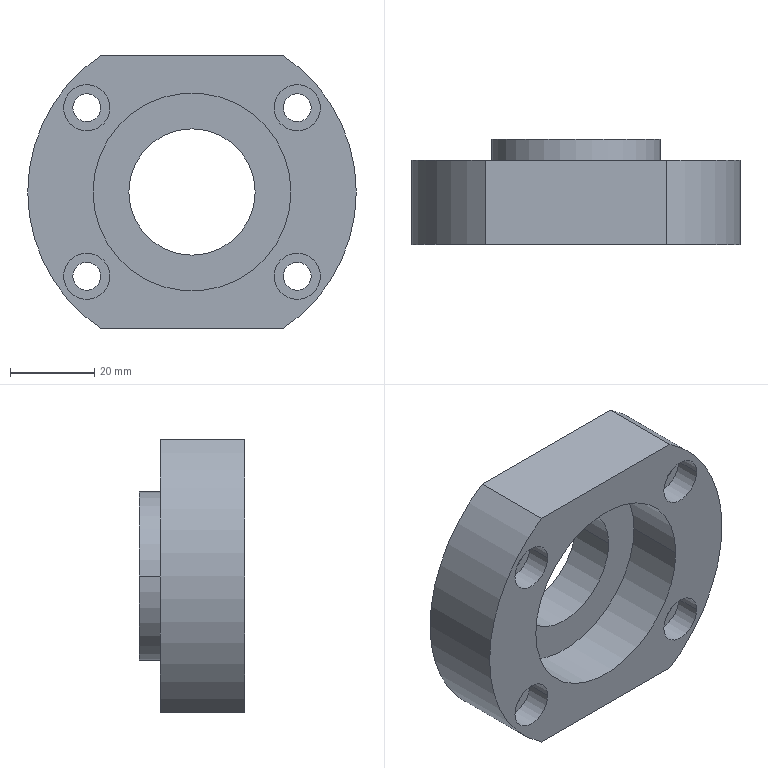Component | SolidWorks | TractionBearingHousing-3 | 1 solid | 35 faces | box 78 x 25 x 65 mm | volume 57981 mm3 | cylinder 25 | plane 10 | commonest cylinder face diameters 11 x8 6.6 x8 78 x3 47 x2 30 x2 40 x2
build123d program:
from build123d import *

# Parameters (mm, degrees)
SKETCH2_W                                       = 19.822
SKETCH2_H                                       = 75.013
EXTRUDE1_DEPTH                                  = 61.556
M6_HEX_SOCKET_HEAD_CAP_SCREW_CBORE1_D           = 6.6
M6_HEX_SOCKET_HEAD_CAP_SCREW_CBORE1_CBORE_D     = 11
M6_HEX_SOCKET_HEAD_CAP_SCREW_CBORE1_CBORE_DEPTH = 6


with BuildPart() as part:
    # Sketch1 → Revolve1 (revolve)
    with BuildSketch(Plane.XY, mode=Mode.PRIVATE) as revolve1_sk:
        Polygon((23.5, 30.807), (39, 30.807), (39, 10.807), (20, 10.807), (20, 5.807), (15, 5.807), (15, 16.807), (23.5, 16.807), align=None)
    revolve(revolve1_sk.sketch.rotate(Axis((0, -994.193, 0), (0, 1, 0)), 90), axis=Axis((0, -994.193, 0), (0, 1, 0)))

    # Sketch2 → Extrude1 (cut, through all)
    with BuildSketch(Plane(origin=(0, 30.807, 0), x_dir=(1, 0, 0), z_dir=(0, 1, 0))):
        with Locations((-42.411, -0.6478)):
            Rectangle(SKETCH2_W, SKETCH2_H)
        with Locations((42.411, -0.6478)):
            Rectangle(SKETCH2_W, SKETCH2_H)
    extrude(amount=-EXTRUDE1_DEPTH, mode=Mode.SUBTRACT)

    # M6 Hex Socket Head Cap Screw CBORE1 (through all)
    with Locations(Plane(origin=(-20, 30.807, -25), x_dir=(0, 0, 1), z_dir=(0, 1, 0))):
        with Locations((0, 0), (0, 40), (50, 40), (50, 0)):
            CounterBoreHole(M6_HEX_SOCKET_HEAD_CAP_SCREW_CBORE1_D / 2, M6_HEX_SOCKET_HEAD_CAP_SCREW_CBORE1_CBORE_D / 2, M6_HEX_SOCKET_HEAD_CAP_SCREW_CBORE1_CBORE_DEPTH)


solid = part.part

# Placed as in the assembly
solid = solid.moved(Location((385.216, 498.79, 59.606), (180, 90, 0)))
STEP:
#1=COLOUR_RGB('',0.7922,0.8196,0.9333);
#2=FILL_AREA_STYLE_COLOUR('',#1);
#3=FILL_AREA_STYLE('',(#2));
#4=SURFACE_STYLE_FILL_AREA(#3);
#5=SURFACE_SIDE_STYLE('',(#4));
#6=SURFACE_STYLE_USAGE(.BOTH.,#5);
#7=PRESENTATION_STYLE_ASSIGNMENT((#6));
#8=CARTESIAN_POINT('',(16.367,18.661,3.134));
#9=VERTEX_POINT('',#8);
#10=CARTESIAN_POINT('',(15.934,18.661,3.134));
#11=VERTEX_POINT('',#10);
#12=CARTESIAN_POINT('',(16.15,18.661,3.134));
#13=DIRECTION('',(0.,-1.,0.));
#14=DIRECTION('',(-1.,0.,0.));
#15=AXIS2_PLACEMENT_3D('',#12,#13,#14);
#16=CIRCLE('',#15,0.2165);
#17=EDGE_CURVE('',#9,#11,#16,.T.);
#18=ORIENTED_EDGE('',*,*,#17,.F.);
#19=CARTESIAN_POINT('',(16.367,18.425,3.134));
#20=VERTEX_POINT('',#19);
#21=CARTESIAN_POINT('',(16.367,18.425,3.134));
#22=DIRECTION('',(0.,-1.,0.));
#23=VECTOR('',#22,39.37);
#24=LINE('',#21,#23);
#25=EDGE_CURVE('',#9,#20,#24,.T.);
#26=ORIENTED_EDGE('',*,*,#25,.T.);
#27=CARTESIAN_POINT('',(15.934,18.425,3.134));
#28=VERTEX_POINT('',#27);
#29=CARTESIAN_POINT('',(16.15,18.425,3.134));
#30=DIRECTION('',(0.,-1.,0.));
#31=DIRECTION('',(-1.,0.,0.));
#32=AXIS2_PLACEMENT_3D('',#29,#30,#31);
#33=CIRCLE('',#32,0.2165);
#34=EDGE_CURVE('',#20,#28,#33,.T.);
#35=ORIENTED_EDGE('',*,*,#34,.T.);
#36=CARTESIAN_POINT('',(15.934,18.425,3.134));
#37=DIRECTION('',(0.,-1.,0.));
#38=VECTOR('',#37,39.37);
#39=LINE('',#36,#38);
#40=EDGE_CURVE('',#11,#28,#39,.T.);
#41=ORIENTED_EDGE('',*,*,#40,.F.);
#42=EDGE_LOOP('',(#18,#26,#35,#41));
#43=FACE_OUTER_BOUND('',#42,.T.);
#44=CARTESIAN_POINT('',(16.15,18.425,3.134));
#45=DIRECTION('',(0.,-1.,0.));
#46=DIRECTION('',(-1.,0.,0.));
#47=AXIS2_PLACEMENT_3D('',#44,#45,#46);
#48=CYLINDRICAL_SURFACE('',#47,0.2165);
#49=ADVANCED_FACE('',(#43),#48,.F.);
#50=CARTESIAN_POINT('',(16.02,19.212,3.134));
#51=VERTEX_POINT('',#50);
#52=CARTESIAN_POINT('',(16.28,19.212,3.134));
#53=VERTEX_POINT('',#52);
#54=CARTESIAN_POINT('',(16.15,19.212,3.134));
#55=DIRECTION('',(-0.,1.,-0.));
#56=DIRECTION('',(1.,0.,0.));
#57=AXIS2_PLACEMENT_3D('',#54,#55,#56);
#58=CIRCLE('',#57,0.1299);
#59=EDGE_CURVE('',#51,#53,#58,.T.);
#60=ORIENTED_EDGE('',*,*,#59,.T.);
#61=CARTESIAN_POINT('',(16.28,18.661,3.134));
#62=VERTEX_POINT('',#61);
#63=CARTESIAN_POINT('',(16.28,18.425,3.134));
#64=DIRECTION('',(0.,-1.,0.));
#65=VECTOR('',#64,39.37);
#66=LINE('',#63,#65);
#67=EDGE_CURVE('',#53,#62,#66,.T.);
#68=ORIENTED_EDGE('',*,*,#67,.T.);
#69=CARTESIAN_POINT('',(16.02,18.661,3.134));
#70=VERTEX_POINT('',#69);
#71=CARTESIAN_POINT('',(16.15,18.661,3.134));
#72=DIRECTION('',(0.,-1.,0.));
#73=DIRECTION('',(-1.,0.,0.));
#74=AXIS2_PLACEMENT_3D('',#71,#72,#73);
#75=CIRCLE('',#74,0.1299);
#76=EDGE_CURVE('',#62,#70,#75,.T.);
#77=ORIENTED_EDGE('',*,*,#76,.T.);
#78=CARTESIAN_POINT('',(16.02,18.425,3.134));
#79=DIRECTION('',(0.,-1.,0.));
#80=VECTOR('',#79,39.37);
#81=LINE('',#78,#80);
#82=EDGE_CURVE('',#51,#70,#81,.T.);
#83=ORIENTED_EDGE('',*,*,#82,.F.);
#84=EDGE_LOOP('',(#60,#68,#77,#83));
#85=FACE_OUTER_BOUND('',#84,.T.);
#86=CARTESIAN_POINT('',(16.15,18.425,3.134));
#87=DIRECTION('',(0.,-1.,0.));
#88=DIRECTION('',(-1.,0.,0.));
#89=AXIS2_PLACEMENT_3D('',#86,#87,#88);
#90=CYLINDRICAL_SURFACE('',#89,0.1299);
#91=ADVANCED_FACE('',(#85),#90,.F.);
#92=CARTESIAN_POINT('',(16.367,18.661,1.559));
#93=VERTEX_POINT('',#92);
#94=CARTESIAN_POINT('',(15.934,18.661,1.559));
#95=VERTEX_POINT('',#94);
#96=CARTESIAN_POINT('',(16.15,18.661,1.559));
#97=DIRECTION('',(0.,-1.,0.));
#98=DIRECTION('',(-1.,0.,0.));
#99=AXIS2_PLACEMENT_3D('',#96,#97,#98);
#100=CIRCLE('',#99,0.2165);
#101=EDGE_CURVE('',#93,#95,#100,.T.);
#102=ORIENTED_EDGE('',*,*,#101,.F.);
#103=CARTESIAN_POINT('',(16.367,18.425,1.559));
#104=VERTEX_POINT('',#103);
#105=CARTESIAN_POINT('',(16.367,18.425,1.559));
#106=DIRECTION('',(0.,-1.,0.));
#107=VECTOR('',#106,39.37);
#108=LINE('',#105,#107);
#109=EDGE_CURVE('',#93,#104,#108,.T.);
#110=ORIENTED_EDGE('',*,*,#109,.T.);
#111=CARTESIAN_POINT('',(15.934,18.425,1.559));
#112=VERTEX_POINT('',#111);
#113=CARTESIAN_POINT('',(16.15,18.425,1.559));
#114=DIRECTION('',(0.,-1.,0.));
#115=DIRECTION('',(-1.,0.,0.));
#116=AXIS2_PLACEMENT_3D('',#113,#114,#115);
#117=CIRCLE('',#116,0.2165);
#118=EDGE_CURVE('',#104,#112,#117,.T.);
#119=ORIENTED_EDGE('',*,*,#118,.T.);
#120=CARTESIAN_POINT('',(15.934,18.425,1.559));
#121=DIRECTION('',(0.,-1.,0.));
#122=VECTOR('',#121,39.37);
#123=LINE('',#120,#122);
#124=EDGE_CURVE('',#95,#112,#123,.T.);
#125=ORIENTED_EDGE('',*,*,#124,.F.);
#126=EDGE_LOOP('',(#102,#110,#119,#125));
#127=FACE_OUTER_BOUND('',#126,.T.);
#128=CARTESIAN_POINT('',(16.15,18.425,1.559));
#129=DIRECTION('',(0.,-1.,0.));
#130=DIRECTION('',(-1.,0.,0.));
#131=AXIS2_PLACEMENT_3D('',#128,#129,#130);
#132=CYLINDRICAL_SURFACE('',#131,0.2165);
#133=ADVANCED_FACE('',(#127),#132,.F.);
#134=CARTESIAN_POINT('',(16.02,19.212,1.559));
#135=VERTEX_POINT('',#134);
#136=CARTESIAN_POINT('',(16.28,19.212,1.559));
#137=VERTEX_POINT('',#136);
#138=CARTESIAN_POINT('',(16.15,19.212,1.559));
#139=DIRECTION('',(-0.,1.,-0.));
#140=DIRECTION('',(1.,0.,0.));
#141=AXIS2_PLACEMENT_3D('',#138,#139,#140);
#142=CIRCLE('',#141,0.1299);
#143=EDGE_CURVE('',#135,#137,#142,.T.);
#144=ORIENTED_EDGE('',*,*,#143,.T.);
#145=CARTESIAN_POINT('',(16.28,18.661,1.559));
#146=VERTEX_POINT('',#145);
#147=CARTESIAN_POINT('',(16.28,18.425,1.559));
#148=DIRECTION('',(0.,-1.,0.));
#149=VECTOR('',#148,39.37);
#150=LINE('',#147,#149);
#151=EDGE_CURVE('',#137,#146,#150,.T.);
#152=ORIENTED_EDGE('',*,*,#151,.T.);
#153=CARTESIAN_POINT('',(16.02,18.661,1.559));
#154=VERTEX_POINT('',#153);
#155=CARTESIAN_POINT('',(16.15,18.661,1.559));
#156=DIRECTION('',(0.,-1.,0.));
#157=DIRECTION('',(-1.,0.,0.));
#158=AXIS2_PLACEMENT_3D('',#155,#156,#157);
#159=CIRCLE('',#158,0.1299);
#160=EDGE_CURVE('',#146,#154,#159,.T.);
#161=ORIENTED_EDGE('',*,*,#160,.T.);
#162=CARTESIAN_POINT('',(16.02,18.425,1.559));
#163=DIRECTION('',(0.,-1.,0.));
#164=VECTOR('',#163,39.37);
#165=LINE('',#162,#164);
#166=EDGE_CURVE('',#135,#154,#165,.T.);
#167=ORIENTED_EDGE('',*,*,#166,.F.);
#168=EDGE_LOOP('',(#144,#152,#161,#167));
#169=FACE_OUTER_BOUND('',#168,.T.);
#170=CARTESIAN_POINT('',(16.15,18.425,1.559));
#171=DIRECTION('',(0.,-1.,0.));
#172=DIRECTION('',(-1.,0.,0.));
#173=AXIS2_PLACEMENT_3D('',#170,#171,#172);
#174=CYLINDRICAL_SURFACE('',#173,0.1299);
#175=ADVANCED_FACE('',(#169),#174,.F.);
#176=CARTESIAN_POINT('',(14.398,18.661,1.559));
#177=VERTEX_POINT('',#176);
#178=CARTESIAN_POINT('',(13.965,18.661,1.559));
#179=VERTEX_POINT('',#178);
#180=CARTESIAN_POINT('',(14.182,18.661,1.559));
#181=DIRECTION('',(0.,-1.,0.));
#182=DIRECTION('',(-1.,0.,0.));
#183=AXIS2_PLACEMENT_3D('',#180,#181,#182);
#184=CIRCLE('',#183,0.2165);
#185=EDGE_CURVE('',#177,#179,#184,.T.);
#186=ORIENTED_EDGE('',*,*,#185,.F.);
#187=CARTESIAN_POINT('',(14.398,18.425,1.559));
#188=VERTEX_POINT('',#187);
#189=CARTESIAN_POINT('',(14.398,18.425,1.559));
#190=DIRECTION('',(0.,-1.,0.));
#191=VECTOR('',#190,39.37);
#192=LINE('',#189,#191);
#193=EDGE_CURVE('',#177,#188,#192,.T.);
#194=ORIENTED_EDGE('',*,*,#193,.T.);
#195=CARTESIAN_POINT('',(13.965,18.425,1.559));
#196=VERTEX_POINT('',#195);
#197=CARTESIAN_POINT('',(14.182,18.425,1.559));
#198=DIRECTION('',(0.,-1.,0.));
#199=DIRECTION('',(-1.,0.,0.));
#200=AXIS2_PLACEMENT_3D('',#197,#198,#199);
#201=CIRCLE('',#200,0.2165);
#202=EDGE_CURVE('',#188,#196,#201,.T.);
#203=ORIENTED_EDGE('',*,*,#202,.T.);
#204=CARTESIAN_POINT('',(13.965,18.425,1.559));
#205=DIRECTION('',(0.,-1.,0.));
#206=VECTOR('',#205,39.37);
#207=LINE('',#204,#206);
#208=EDGE_CURVE('',#179,#196,#207,.T.);
#209=ORIENTED_EDGE('',*,*,#208,.F.);
#210=EDGE_LOOP('',(#186,#194,#203,#209));
#211=FACE_OUTER_BOUND('',#210,.T.);
#212=CARTESIAN_POINT('',(14.182,18.425,1.559));
#213=DIRECTION('',(0.,-1.,0.));
#214=DIRECTION('',(-1.,0.,0.));
#215=AXIS2_PLACEMENT_3D('',#212,#213,#214);
#216=CYLINDRICAL_SURFACE('',#215,0.2165);
#217=ADVANCED_FACE('',(#211),#216,.F.);
#218=CARTESIAN_POINT('',(14.052,19.212,1.559));
#219=VERTEX_POINT('',#218);
#220=CARTESIAN_POINT('',(14.312,19.212,1.559));
#221=VERTEX_POINT('',#220);
#222=CARTESIAN_POINT('',(14.182,19.212,1.559));
#223=DIRECTION('',(-0.,1.,-0.));
#224=DIRECTION('',(1.,0.,0.));
#225=AXIS2_PLACEMENT_3D('',#222,#223,#224);
#226=CIRCLE('',#225,0.1299);
#227=EDGE_CURVE('',#219,#221,#226,.T.);
#228=ORIENTED_EDGE('',*,*,#227,.T.);
#229=CARTESIAN_POINT('',(14.312,18.661,1.559));
#230=VERTEX_POINT('',#229);
#231=CARTESIAN_POINT('',(14.312,18.425,1.559));
#232=DIRECTION('',(0.,-1.,0.));
#233=VECTOR('',#232,39.37);
#234=LINE('',#231,#233);
#235=EDGE_CURVE('',#221,#230,#234,.T.);
#236=ORIENTED_EDGE('',*,*,#235,.T.);
#237=CARTESIAN_POINT('',(14.052,18.661,1.559));
#238=VERTEX_POINT('',#237);
#239=CARTESIAN_POINT('',(14.182,18.661,1.559));
#240=DIRECTION('',(0.,-1.,0.));
#241=DIRECTION('',(-1.,0.,0.));
#242=AXIS2_PLACEMENT_3D('',#239,#240,#241);
#243=CIRCLE('',#242,0.1299);
#244=EDGE_CURVE('',#230,#238,#243,.T.);
#245=ORIENTED_EDGE('',*,*,#244,.T.);
#246=CARTESIAN_POINT('',(14.052,18.425,1.559));
#247=DIRECTION('',(0.,-1.,0.));
#248=VECTOR('',#247,39.37);
#249=LINE('',#246,#248);
#250=EDGE_CURVE('',#219,#238,#249,.T.);
#251=ORIENTED_EDGE('',*,*,#250,.F.);
#252=EDGE_LOOP('',(#228,#236,#245,#251));
#253=FACE_OUTER_BOUND('',#252,.T.);
#254=CARTESIAN_POINT('',(14.182,18.425,1.559));
#255=DIRECTION('',(0.,-1.,0.));
#256=DIRECTION('',(-1.,0.,0.));
#257=AXIS2_PLACEMENT_3D('',#254,#255,#256);
#258=CYLINDRICAL_SURFACE('',#257,0.1299);
#259=ADVANCED_FACE('',(#253),#258,.F.);
#260=CARTESIAN_POINT('',(14.398,18.661,3.134));
#261=VERTEX_POINT('',#260);
#262=CARTESIAN_POINT('',(13.965,18.661,3.134));
#263=VERTEX_POINT('',#262);
#264=CARTESIAN_POINT('',(14.182,18.661,3.134));
#265=DIRECTION('',(0.,-1.,0.));
#266=DIRECTION('',(-1.,0.,0.));
#267=AXIS2_PLACEMENT_3D('',#264,#265,#266);
#268=CIRCLE('',#267,0.2165);
#269=EDGE_CURVE('',#261,#263,#268,.T.);
#270=ORIENTED_EDGE('',*,*,#269,.F.);
#271=CARTESIAN_POINT('',(14.398,18.425,3.134));
#272=VERTEX_POINT('',#271);
#273=CARTESIAN_POINT('',(14.398,18.425,3.134));
#274=DIRECTION('',(0.,-1.,0.));
#275=VECTOR('',#274,39.37);
#276=LINE('',#273,#275);
#277=EDGE_CURVE('',#261,#272,#276,.T.);
#278=ORIENTED_EDGE('',*,*,#277,.T.);
#279=CARTESIAN_POINT('',(13.965,18.425,3.134));
#280=VERTEX_POINT('',#279);
#281=CARTESIAN_POINT('',(14.182,18.425,3.134));
#282=DIRECTION('',(0.,-1.,0.));
#283=DIRECTION('',(-1.,0.,0.));
#284=AXIS2_PLACEMENT_3D('',#281,#282,#283);
#285=CIRCLE('',#284,0.2165);
#286=EDGE_CURVE('',#272,#280,#285,.T.);
#287=ORIENTED_EDGE('',*,*,#286,.T.);
#288=CARTESIAN_POINT('',(13.965,18.425,3.134));
#289=DIRECTION('',(0.,-1.,0.));
#290=VECTOR('',#289,39.37);
#291=LINE('',#288,#290);
#292=EDGE_CURVE('',#263,#280,#291,.T.);
#293=ORIENTED_EDGE('',*,*,#292,.F.);
#294=EDGE_LOOP('',(#270,#278,#287,#293));
#295=FACE_OUTER_BOUND('',#294,.T.);
#296=CARTESIAN_POINT('',(14.182,18.425,3.134));
#297=DIRECTION('',(0.,-1.,0.));
#298=DIRECTION('',(-1.,0.,0.));
#299=AXIS2_PLACEMENT_3D('',#296,#297,#298);
#300=CYLINDRICAL_SURFACE('',#299,0.2165);
#301=ADVANCED_FACE('',(#295),#300,.F.);
#302=CARTESIAN_POINT('',(14.052,19.212,3.134));
#303=VERTEX_POINT('',#302);
#304=CARTESIAN_POINT('',(14.312,19.212,3.134));
#305=VERTEX_POINT('',#304);
#306=CARTESIAN_POINT('',(14.182,19.212,3.134));
#307=DIRECTION('',(-0.,1.,-0.));
#308=DIRECTION('',(1.,0.,0.));
#309=AXIS2_PLACEMENT_3D('',#306,#307,#308);
#310=CIRCLE('',#309,0.1299);
#311=EDGE_CURVE('',#303,#305,#310,.T.);
#312=ORIENTED_EDGE('',*,*,#311,.T.);
#313=CARTESIAN_POINT('',(14.312,18.661,3.134));
#314=VERTEX_POINT('',#313);
#315=CARTESIAN_POINT('',(14.312,18.425,3.134));
#316=DIRECTION('',(0.,-1.,0.));
#317=VECTOR('',#316,39.37);
#318=LINE('',#315,#317);
#319=EDGE_CURVE('',#305,#314,#318,.T.);
#320=ORIENTED_EDGE('',*,*,#319,.T.);
#321=CARTESIAN_POINT('',(14.052,18.661,3.134));
#322=VERTEX_POINT('',#321);
#323=CARTESIAN_POINT('',(14.182,18.661,3.134));
#324=DIRECTION('',(0.,-1.,0.));
#325=DIRECTION('',(-1.,0.,0.));
#326=AXIS2_PLACEMENT_3D('',#323,#324,#325);
#327=CIRCLE('',#326,0.1299);
#328=EDGE_CURVE('',#314,#322,#327,.T.);
#329=ORIENTED_EDGE('',*,*,#328,.T.);
#330=CARTESIAN_POINT('',(14.052,18.425,3.134));
#331=DIRECTION('',(0.,-1.,0.));
#332=VECTOR('',#331,39.37);
#333=LINE('',#330,#332);
#334=EDGE_CURVE('',#303,#322,#333,.T.);
#335=ORIENTED_EDGE('',*,*,#334,.F.);
#336=EDGE_LOOP('',(#312,#320,#329,#335));
#337=FACE_OUTER_BOUND('',#336,.T.);
#338=CARTESIAN_POINT('',(14.182,18.425,3.134));
#339=DIRECTION('',(0.,-1.,0.));
#340=DIRECTION('',(-1.,0.,0.));
#341=AXIS2_PLACEMENT_3D('',#338,#339,#340);
#342=CYLINDRICAL_SURFACE('',#341,0.1299);
#343=ADVANCED_FACE('',(#337),#342,.F.);
#344=CARTESIAN_POINT('',(14.241,18.425,2.347));
#345=VERTEX_POINT('',#344);
#346=CARTESIAN_POINT('',(16.091,18.425,2.347));
#347=VERTEX_POINT('',#346);
#348=CARTESIAN_POINT('',(15.166,18.425,2.347));
#349=DIRECTION('',(-0.,1.,-0.));
#350=DIRECTION('',(1.,0.,0.));
#351=AXIS2_PLACEMENT_3D('',#348,#349,#350);
#352=CIRCLE('',#351,0.9252);
#353=EDGE_CURVE('',#345,#347,#352,.T.);
#354=ORIENTED_EDGE('',*,*,#353,.F.);
#355=CARTESIAN_POINT('',(14.241,18.976,2.347));
#356=VERTEX_POINT('',#355);
#357=CARTESIAN_POINT('',(14.241,58.779,2.347));
#358=DIRECTION('',(-0.,1.,-0.));
#359=VECTOR('',#358,39.37);
#360=LINE('',#357,#359);
#361=EDGE_CURVE('',#345,#356,#360,.T.);
#362=ORIENTED_EDGE('',*,*,#361,.T.);
#363=CARTESIAN_POINT('',(16.091,18.976,2.347));
#364=VERTEX_POINT('',#363);
#365=CARTESIAN_POINT('',(15.166,18.976,2.347));
#366=DIRECTION('',(-0.,1.,-0.));
#367=DIRECTION('',(1.,0.,0.));
#368=AXIS2_PLACEMENT_3D('',#365,#366,#367);
#369=CIRCLE('',#368,0.9252);
#370=EDGE_CURVE('',#356,#364,#369,.T.);
#371=ORIENTED_EDGE('',*,*,#370,.T.);
#372=CARTESIAN_POINT('',(16.091,58.779,2.347));
#373=DIRECTION('',(-0.,1.,-0.));
#374=VECTOR('',#373,39.37);
#375=LINE('',#372,#374);
#376=EDGE_CURVE('',#347,#364,#375,.T.);
#377=ORIENTED_EDGE('',*,*,#376,.F.);
#378=EDGE_LOOP('',(#354,#362,#371,#377));
#379=FACE_OUTER_BOUND('',#378,.T.);
#380=CARTESIAN_POINT('',(15.166,58.779,2.347));
#381=DIRECTION('',(-0.,1.,-0.));
#382=DIRECTION('',(1.,0.,0.));
#383=AXIS2_PLACEMENT_3D('',#380,#381,#382);
#384=CYLINDRICAL_SURFACE('',#383,0.9252);
#385=ADVANCED_FACE('',(#379),#384,.F.);
#386=CARTESIAN_POINT('',(14.575,18.976,2.347));
#387=VERTEX_POINT('',#386);
#388=CARTESIAN_POINT('',(15.757,18.976,2.347));
#389=VERTEX_POINT('',#388);
#390=CARTESIAN_POINT('',(15.166,18.976,2.347));
#391=DIRECTION('',(-0.,1.,-0.));
#392=DIRECTION('',(1.,0.,0.));
#393=AXIS2_PLACEMENT_3D('',#390,#391,#392);
#394=CIRCLE('',#393,0.5906);
#395=EDGE_CURVE('',#387,#389,#394,.T.);
#396=ORIENTED_EDGE('',*,*,#395,.F.);
#397=CARTESIAN_POINT('',(14.575,19.409,2.347));
#398=VERTEX_POINT('',#397);
#399=CARTESIAN_POINT('',(14.575,58.779,2.347));
#400=DIRECTION('',(-0.,1.,-0.));
#401=VECTOR('',#400,39.37);
#402=LINE('',#399,#401);
#403=EDGE_CURVE('',#387,#398,#402,.T.);
#404=ORIENTED_EDGE('',*,*,#403,.T.);
#405=CARTESIAN_POINT('',(15.757,19.409,2.347));
#406=VERTEX_POINT('',#405);
#407=CARTESIAN_POINT('',(15.166,19.409,2.347));
#408=DIRECTION('',(-0.,1.,-0.));
#409=DIRECTION('',(1.,0.,0.));
#410=AXIS2_PLACEMENT_3D('',#407,#408,#409);
#411=CIRCLE('',#410,0.5906);
#412=EDGE_CURVE('',#398,#406,#411,.T.);
#413=ORIENTED_EDGE('',*,*,#412,.T.);
#414=CARTESIAN_POINT('',(15.757,58.779,2.347));
#415=DIRECTION('',(-0.,1.,-0.));
#416=VECTOR('',#415,39.37);
#417=LINE('',#414,#416);
#418=EDGE_CURVE('',#389,#406,#417,.T.);
#419=ORIENTED_EDGE('',*,*,#418,.F.);
#420=EDGE_LOOP('',(#396,#404,#413,#419));
#421=FACE_OUTER_BOUND('',#420,.T.);
#422=CARTESIAN_POINT('',(15.166,58.779,2.347));
#423=DIRECTION('',(-0.,1.,-0.));
#424=DIRECTION('',(1.,0.,0.));
#425=AXIS2_PLACEMENT_3D('',#422,#423,#424);
#426=CYLINDRICAL_SURFACE('',#425,0.5906);
#427=ADVANCED_FACE('',(#421),#426,.F.);
#428=CARTESIAN_POINT('',(15.953,19.212,2.347));
#429=VERTEX_POINT('',#428);
#430=CARTESIAN_POINT('',(14.379,19.212,2.347));
#431=VERTEX_POINT('',#430);
#432=CARTESIAN_POINT('',(15.166,19.212,2.347));
#433=DIRECTION('',(-0.,1.,-0.));
#434=DIRECTION('',(1.,0.,0.));
#435=AXIS2_PLACEMENT_3D('',#432,#433,#434);
#436=CIRCLE('',#435,0.7874);
#437=EDGE_CURVE('',#429,#431,#436,.T.);
#438=ORIENTED_EDGE('',*,*,#437,.T.);
#439=CARTESIAN_POINT('',(14.379,19.409,2.347));
#440=VERTEX_POINT('',#439);
#441=CARTESIAN_POINT('',(14.379,58.779,2.347));
#442=DIRECTION('',(-0.,1.,-0.));
#443=VECTOR('',#442,39.37);
#444=LINE('',#441,#443);
#445=EDGE_CURVE('',#431,#440,#444,.T.);
#446=ORIENTED_EDGE('',*,*,#445,.T.);
#447=CARTESIAN_POINT('',(15.953,19.409,2.347));
#448=VERTEX_POINT('',#447);
#449=CARTESIAN_POINT('',(15.166,19.409,2.347));
#450=DIRECTION('',(-0.,1.,-0.));
#451=DIRECTION('',(1.,0.,0.));
#452=AXIS2_PLACEMENT_3D('',#449,#450,#451);
#453=CIRCLE('',#452,0.7874);
#454=EDGE_CURVE('',#448,#440,#453,.T.);
#455=ORIENTED_EDGE('',*,*,#454,.F.);
#456=CARTESIAN_POINT('',(15.953,58.779,2.347));
#457=DIRECTION('',(-0.,1.,-0.));
#458=VECTOR('',#457,39.37);
#459=LINE('',#456,#458);
#460=EDGE_CURVE('',#429,#448,#459,.T.);
#461=ORIENTED_EDGE('',*,*,#460,.F.);
#462=EDGE_LOOP('',(#438,#446,#455,#461));
#463=FACE_OUTER_BOUND('',#462,.T.);
#464=CARTESIAN_POINT('',(15.166,58.779,2.347));
#465=DIRECTION('',(-0.,1.,-0.));
#466=DIRECTION('',(1.,0.,0.));
#467=AXIS2_PLACEMENT_3D('',#464,#465,#466);
#468=CYLINDRICAL_SURFACE('',#467,0.7874);
#469=ADVANCED_FACE('',(#463),#468,.T.);
#470=CARTESIAN_POINT('',(16.015,18.425,3.626));
#471=VERTEX_POINT('',#470);
#472=CARTESIAN_POINT('',(16.701,18.425,2.347));
#473=VERTEX_POINT('',#472);
#474=CARTESIAN_POINT('',(15.166,18.425,2.347));
#475=DIRECTION('',(-0.,1.,-0.));
#476=DIRECTION('',(1.,0.,0.));
#477=AXIS2_PLACEMENT_3D('',#474,#475,#476);
#478=CIRCLE('',#477,1.535);
#479=EDGE_CURVE('',#471,#473,#478,.T.);
#480=ORIENTED_EDGE('',*,*,#479,.T.);
#481=CARTESIAN_POINT('',(16.701,19.212,2.347));
#482=VERTEX_POINT('',#481);
#483=CARTESIAN_POINT('',(16.701,58.779,2.347));
#484=DIRECTION('',(-0.,1.,-0.));
#485=VECTOR('',#484,39.37);
#486=LINE('',#483,#485);
#487=EDGE_CURVE('',#473,#482,#486,.T.);
#488=ORIENTED_EDGE('',*,*,#487,.T.);
#489=CARTESIAN_POINT('',(16.015,19.212,3.626));
#490=VERTEX_POINT('',#489);
#491=CARTESIAN_POINT('',(15.166,19.212,2.347));
#492=DIRECTION('',(-0.,1.,-0.));
#493=DIRECTION('',(1.,0.,0.));
#494=AXIS2_PLACEMENT_3D('',#491,#492,#493);
#495=CIRCLE('',#494,1.535);
#496=EDGE_CURVE('',#490,#482,#495,.T.);
#497=ORIENTED_EDGE('',*,*,#496,.F.);
#498=CARTESIAN_POINT('',(16.015,58.779,3.626));
#499=DIRECTION('',(-0.,1.,-0.));
#500=VECTOR('',#499,39.37);
#501=LINE('',#498,#500);
#502=EDGE_CURVE('',#471,#490,#501,.T.);
#503=ORIENTED_EDGE('',*,*,#502,.F.);
#504=EDGE_LOOP('',(#480,#488,#497,#503));
#505=FACE_OUTER_BOUND('',#504,.T.);
#506=CARTESIAN_POINT('',(15.166,58.779,2.347));
#507=DIRECTION('',(-0.,1.,-0.));
#508=DIRECTION('',(1.,0.,0.));
#509=AXIS2_PLACEMENT_3D('',#506,#507,#508);
#510=CYLINDRICAL_SURFACE('',#509,1.535);
#511=ADVANCED_FACE('',(#505),#510,.T.);
#512=ORIENTED_EDGE('',*,*,#487,.F.);
#513=CARTESIAN_POINT('',(16.015,18.425,1.067));
#514=VERTEX_POINT('',#513);
#515=CARTESIAN_POINT('',(15.166,18.425,2.347));
#516=DIRECTION('',(-0.,1.,-0.));
#517=DIRECTION('',(1.,0.,0.));
#518=AXIS2_PLACEMENT_3D('',#515,#516,#517);
#519=CIRCLE('',#518,1.535);
#520=EDGE_CURVE('',#473,#514,#519,.T.);
#521=ORIENTED_EDGE('',*,*,#520,.T.);
#522=CARTESIAN_POINT('',(16.015,19.212,1.067));
#523=VERTEX_POINT('',#522);
#524=CARTESIAN_POINT('',(16.015,58.779,1.067));
#525=DIRECTION('',(0.,-1.,0.));
#526=VECTOR('',#525,39.37);
#527=LINE('',#524,#526);
#528=EDGE_CURVE('',#523,#514,#527,.T.);
#529=ORIENTED_EDGE('',*,*,#528,.F.);
#530=CARTESIAN_POINT('',(15.166,19.212,2.347));
#531=DIRECTION('',(-0.,1.,-0.));
#532=DIRECTION('',(1.,0.,0.));
#533=AXIS2_PLACEMENT_3D('',#530,#531,#532);
#534=CIRCLE('',#533,1.535);
#535=EDGE_CURVE('',#482,#523,#534,.T.);
#536=ORIENTED_EDGE('',*,*,#535,.F.);
#537=EDGE_LOOP('',(#512,#521,#529,#536));
#538=FACE_OUTER_BOUND('',#537,.T.);
#539=CARTESIAN_POINT('',(15.166,58.779,2.347));
#540=DIRECTION('',(-0.,1.,-0.));
#541=DIRECTION('',(1.,0.,0.));
#542=AXIS2_PLACEMENT_3D('',#539,#540,#541);
#543=CYLINDRICAL_SURFACE('',#542,1.535);
#544=ADVANCED_FACE('',(#538),#543,.T.);
#545=CARTESIAN_POINT('',(14.317,18.425,1.067));
#546=VERTEX_POINT('',#545);
#547=CARTESIAN_POINT('',(14.317,19.212,1.067));
#548=VERTEX_POINT('',#547);
#549=CARTESIAN_POINT('',(14.317,58.779,1.067));
#550=DIRECTION('',(-0.,1.,-0.));
#551=VECTOR('',#550,39.37);
#552=LINE('',#549,#551);
#553=EDGE_CURVE('',#546,#548,#552,.T.);
#554=ORIENTED_EDGE('',*,*,#553,.F.);
#555=CARTESIAN_POINT('',(14.317,18.425,3.626));
#556=VERTEX_POINT('',#555);
#557=CARTESIAN_POINT('',(15.166,18.425,2.347));
#558=DIRECTION('',(-0.,1.,-0.));
#559=DIRECTION('',(1.,0.,0.));
#560=AXIS2_PLACEMENT_3D('',#557,#558,#559);
#561=CIRCLE('',#560,1.535);
#562=EDGE_CURVE('',#546,#556,#561,.T.);
#563=ORIENTED_EDGE('',*,*,#562,.T.);
#564=CARTESIAN_POINT('',(14.317,19.212,3.626));
#565=VERTEX_POINT('',#564);
#566=CARTESIAN_POINT('',(14.317,58.779,3.626));
#567=DIRECTION('',(0.,-1.,0.));
#568=VECTOR('',#567,39.37);
#569=LINE('',#566,#568);
#570=EDGE_CURVE('',#565,#556,#569,.T.);
#571=ORIENTED_EDGE('',*,*,#570,.F.);
#572=CARTESIAN_POINT('',(15.166,19.212,2.347));
#573=DIRECTION('',(-0.,1.,-0.));
#574=DIRECTION('',(1.,0.,0.));
#575=AXIS2_PLACEMENT_3D('',#572,#573,#574);
#576=CIRCLE('',#575,1.535);
#577=EDGE_CURVE('',#548,#565,#576,.T.);
#578=ORIENTED_EDGE('',*,*,#577,.F.);
#579=EDGE_LOOP('',(#554,#563,#571,#578));
#580=FACE_OUTER_BOUND('',#579,.T.);
#581=CARTESIAN_POINT('',(15.166,58.779,2.347));
#582=DIRECTION('',(-0.,1.,-0.));
#583=DIRECTION('',(1.,0.,0.));
#584=AXIS2_PLACEMENT_3D('',#581,#582,#583);
#585=CYLINDRICAL_SURFACE('',#584,1.535);
#586=ADVANCED_FACE('',(#580),#585,.T.);
#587=ORIENTED_EDGE('',*,*,#59,.F.);
#588=CARTESIAN_POINT('',(16.15,19.212,3.134));
#589=DIRECTION('',(-0.,1.,-0.));
#590=DIRECTION('',(1.,0.,0.));
#591=AXIS2_PLACEMENT_3D('',#588,#589,#590);
#592=CIRCLE('',#591,0.1299);
#593=EDGE_CURVE('',#53,#51,#592,.T.);
#594=ORIENTED_EDGE('',*,*,#593,.F.);
#595=EDGE_LOOP('',(#587,#594));
#596=FACE_BOUND('',#595,.T.);
#597=ORIENTED_EDGE('',*,*,#143,.F.);
#598=CARTESIAN_POINT('',(16.15,19.212,1.559));
#599=DIRECTION('',(-0.,1.,-0.));
#600=DIRECTION('',(1.,0.,0.));
#601=AXIS2_PLACEMENT_3D('',#598,#599,#600);
#602=CIRCLE('',#601,0.1299);
#603=EDGE_CURVE('',#137,#135,#602,.T.);
#604=ORIENTED_EDGE('',*,*,#603,.F.);
#605=EDGE_LOOP('',(#597,#604));
#606=FACE_BOUND('',#605,.T.);
#607=ORIENTED_EDGE('',*,*,#227,.F.);
#608=CARTESIAN_POINT('',(14.182,19.212,1.559));
#609=DIRECTION('',(-0.,1.,-0.));
#610=DIRECTION('',(1.,0.,0.));
#611=AXIS2_PLACEMENT_3D('',#608,#609,#610);
#612=CIRCLE('',#611,0.1299);
#613=EDGE_CURVE('',#221,#219,#612,.T.);
#614=ORIENTED_EDGE('',*,*,#613,.F.);
#615=EDGE_LOOP('',(#607,#614));
#616=FACE_BOUND('',#615,.T.);
#617=ORIENTED_EDGE('',*,*,#311,.F.);
#618=CARTESIAN_POINT('',(14.182,19.212,3.134));
#619=DIRECTION('',(-0.,1.,-0.));
#620=DIRECTION('',(1.,0.,0.));
#621=AXIS2_PLACEMENT_3D('',#618,#619,#620);
#622=CIRCLE('',#621,0.1299);
#623=EDGE_CURVE('',#305,#303,#622,.T.);
#624=ORIENTED_EDGE('',*,*,#623,.F.);
#625=EDGE_LOOP('',(#617,#624));
#626=FACE_BOUND('',#625,.T.);
#627=CARTESIAN_POINT('',(15.166,19.212,1.067));
#628=DIRECTION('',(1.,0.,-0.));
#629=VECTOR('',#628,39.37);
#630=LINE('',#627,#629);
#631=EDGE_CURVE('',#548,#523,#630,.T.);
#632=ORIENTED_EDGE('',*,*,#631,.F.);
#633=ORIENTED_EDGE('',*,*,#577,.T.);
#634=CARTESIAN_POINT('',(15.166,19.212,3.626));
#635=DIRECTION('',(-1.,-0.,-0.));
#636=VECTOR('',#635,39.37);
#637=LINE('',#634,#636);
#638=EDGE_CURVE('',#490,#565,#637,.T.);
#639=ORIENTED_EDGE('',*,*,#638,.F.);
#640=ORIENTED_EDGE('',*,*,#496,.T.);
#641=ORIENTED_EDGE('',*,*,#535,.T.);
#642=EDGE_LOOP('',(#632,#633,#639,#640,#641));
#643=FACE_OUTER_BOUND('',#642,.T.);
#644=ORIENTED_EDGE('',*,*,#437,.F.);
#645=CARTESIAN_POINT('',(15.166,19.212,2.347));
#646=DIRECTION('',(-0.,1.,-0.));
#647=DIRECTION('',(1.,0.,0.));
#648=AXIS2_PLACEMENT_3D('',#645,#646,#647);
#649=CIRCLE('',#648,0.7874);
#650=EDGE_CURVE('',#431,#429,#649,.T.);
#651=ORIENTED_EDGE('',*,*,#650,.F.);
#652=EDGE_LOOP('',(#644,#651));
#653=FACE_BOUND('',#652,.T.);
#654=CARTESIAN_POINT('',(15.166,19.212,0.8113));
#655=DIRECTION('',(-0.,1.,-0.));
#656=DIRECTION('',(1.,0.,-0.));
#657=AXIS2_PLACEMENT_3D('',#654,#655,#656);
#658=PLANE('',#657);
#659=ADVANCED_FACE('',(#596,#606,#616,#626,#643,#653),#658,.T.);
#660=ORIENTED_EDGE('',*,*,#445,.F.);
#661=ORIENTED_EDGE('',*,*,#650,.T.);
#662=ORIENTED_EDGE('',*,*,#460,.T.);
#663=CARTESIAN_POINT('',(15.166,19.409,2.347));
#664=DIRECTION('',(-0.,1.,-0.));
#665=DIRECTION('',(1.,0.,0.));
#666=AXIS2_PLACEMENT_3D('',#663,#664,#665);
#667=CIRCLE('',#666,0.7874);
#668=EDGE_CURVE('',#440,#448,#667,.T.);
#669=ORIENTED_EDGE('',*,*,#668,.F.);
#670=EDGE_LOOP('',(#660,#661,#662,#669));
#671=FACE_OUTER_BOUND('',#670,.T.);
#672=CARTESIAN_POINT('',(15.166,58.779,2.347));
#673=DIRECTION('',(-0.,1.,-0.));
#674=DIRECTION('',(1.,0.,0.));
#675=AXIS2_PLACEMENT_3D('',#672,#673,#674);
#676=CYLINDRICAL_SURFACE('',#675,0.7874);
#677=ADVANCED_FACE('',(#671),#676,.T.);
#678=ORIENTED_EDGE('',*,*,#454,.T.);
#679=ORIENTED_EDGE('',*,*,#668,.T.);
#680=EDGE_LOOP('',(#678,#679));
#681=FACE_OUTER_BOUND('',#680,.T.);
#682=CARTESIAN_POINT('',(15.166,19.409,2.347));
#683=DIRECTION('',(-0.,1.,-0.));
#684=DIRECTION('',(1.,0.,0.));
#685=AXIS2_PLACEMENT_3D('',#682,#683,#684);
#686=CIRCLE('',#685,0.5906);
#687=EDGE_CURVE('',#406,#398,#686,.T.);
#688=ORIENTED_EDGE('',*,*,#687,.F.);
#689=ORIENTED_EDGE('',*,*,#412,.F.);
#690=EDGE_LOOP('',(#688,#689));
#691=FACE_BOUND('',#690,.T.);
#692=CARTESIAN_POINT('',(15.166,19.409,1.559));
#693=DIRECTION('',(-0.,1.,-0.));
#694=DIRECTION('',(1.,0.,-0.));
#695=AXIS2_PLACEMENT_3D('',#692,#693,#694);
#696=PLANE('',#695);
#697=ADVANCED_FACE('',(#681,#691),#696,.T.);
#698=ORIENTED_EDGE('',*,*,#403,.F.);
#699=CARTESIAN_POINT('',(15.166,18.976,2.347));
#700=DIRECTION('',(-0.,1.,-0.));
#701=DIRECTION('',(1.,0.,0.));
#702=AXIS2_PLACEMENT_3D('',#699,#700,#701);
#703=CIRCLE('',#702,0.5906);
#704=EDGE_CURVE('',#389,#387,#703,.T.);
#705=ORIENTED_EDGE('',*,*,#704,.F.);
#706=ORIENTED_EDGE('',*,*,#418,.T.);
#707=ORIENTED_EDGE('',*,*,#687,.T.);
#708=EDGE_LOOP('',(#698,#705,#706,#707));
#709=FACE_OUTER_BOUND('',#708,.T.);
#710=CARTESIAN_POINT('',(15.166,58.779,2.347));
#711=DIRECTION('',(-0.,1.,-0.));
#712=DIRECTION('',(1.,0.,0.));
#713=AXIS2_PLACEMENT_3D('',#710,#711,#712);
#714=CYLINDRICAL_SURFACE('',#713,0.5906);
#715=ADVANCED_FACE('',(#709),#714,.F.);
#716=ORIENTED_EDGE('',*,*,#704,.T.);
#717=ORIENTED_EDGE('',*,*,#395,.T.);
#718=EDGE_LOOP('',(#716,#717));
#719=FACE_BOUND('',#718,.T.);
#720=CARTESIAN_POINT('',(15.166,18.976,2.347));
#721=DIRECTION('',(-0.,1.,-0.));
#722=DIRECTION('',(1.,0.,0.));
#723=AXIS2_PLACEMENT_3D('',#720,#721,#722);
#724=CIRCLE('',#723,0.9252);
#725=EDGE_CURVE('',#364,#356,#724,.T.);
#726=ORIENTED_EDGE('',*,*,#725,.F.);
#727=ORIENTED_EDGE('',*,*,#370,.F.);
#728=EDGE_LOOP('',(#726,#727));
#729=FACE_OUTER_BOUND('',#728,.T.);
#730=CARTESIAN_POINT('',(15.166,18.976,1.421));
#731=DIRECTION('',(0.,-1.,0.));
#732=DIRECTION('',(-1.,-0.,0.));
#733=AXIS2_PLACEMENT_3D('',#730,#731,#732);
#734=PLANE('',#733);
#735=ADVANCED_FACE('',(#719,#729),#734,.T.);
#736=ORIENTED_EDGE('',*,*,#361,.F.);
#737=CARTESIAN_POINT('',(15.166,18.425,2.347));
#738=DIRECTION('',(-0.,1.,-0.));
#739=DIRECTION('',(1.,0.,0.));
#740=AXIS2_PLACEMENT_3D('',#737,#738,#739);
#741=CIRCLE('',#740,0.9252);
#742=EDGE_CURVE('',#347,#345,#741,.T.);
#743=ORIENTED_EDGE('',*,*,#742,.F.);
#744=ORIENTED_EDGE('',*,*,#376,.T.);
#745=ORIENTED_EDGE('',*,*,#725,.T.);
#746=EDGE_LOOP('',(#736,#743,#744,#745));
#747=FACE_OUTER_BOUND('',#746,.T.);
#748=CARTESIAN_POINT('',(15.166,58.779,2.347));
#749=DIRECTION('',(-0.,1.,-0.));
#750=DIRECTION('',(1.,0.,0.));
#751=AXIS2_PLACEMENT_3D('',#748,#749,#750);
#752=CYLINDRICAL_SURFACE('',#751,0.9252);
#753=ADVANCED_FACE('',(#747),#752,.F.);
#754=CARTESIAN_POINT('',(16.15,18.425,3.134));
#755=DIRECTION('',(0.,-1.,0.));
#756=DIRECTION('',(-1.,0.,0.));
#757=AXIS2_PLACEMENT_3D('',#754,#755,#756);
#758=CIRCLE('',#757,0.2165);
#759=EDGE_CURVE('',#28,#20,#758,.T.);
#760=ORIENTED_EDGE('',*,*,#759,.F.);
#761=ORIENTED_EDGE('',*,*,#34,.F.);
#762=EDGE_LOOP('',(#760,#761));
#763=FACE_BOUND('',#762,.T.);
#764=CARTESIAN_POINT('',(16.15,18.425,1.559));
#765=DIRECTION('',(0.,-1.,0.));
#766=DIRECTION('',(-1.,0.,0.));
#767=AXIS2_PLACEMENT_3D('',#764,#765,#766);
#768=CIRCLE('',#767,0.2165);
#769=EDGE_CURVE('',#112,#104,#768,.T.);
#770=ORIENTED_EDGE('',*,*,#769,.F.);
#771=ORIENTED_EDGE('',*,*,#118,.F.);
#772=EDGE_LOOP('',(#770,#771));
#773=FACE_BOUND('',#772,.T.);
#774=CARTESIAN_POINT('',(14.182,18.425,1.559));
#775=DIRECTION('',(0.,-1.,0.));
#776=DIRECTION('',(-1.,0.,0.));
#777=AXIS2_PLACEMENT_3D('',#774,#775,#776);
#778=CIRCLE('',#777,0.2165);
#779=EDGE_CURVE('',#196,#188,#778,.T.);
#780=ORIENTED_EDGE('',*,*,#779,.F.);
#781=ORIENTED_EDGE('',*,*,#202,.F.);
#782=EDGE_LOOP('',(#780,#781));
#783=FACE_BOUND('',#782,.T.);
#784=CARTESIAN_POINT('',(14.182,18.425,3.134));
#785=DIRECTION('',(0.,-1.,0.));
#786=DIRECTION('',(-1.,0.,0.));
#787=AXIS2_PLACEMENT_3D('',#784,#785,#786);
#788=CIRCLE('',#787,0.2165);
#789=EDGE_CURVE('',#280,#272,#788,.T.);
#790=ORIENTED_EDGE('',*,*,#789,.F.);
#791=ORIENTED_EDGE('',*,*,#286,.F.);
#792=EDGE_LOOP('',(#790,#791));
#793=FACE_BOUND('',#792,.T.);
#794=CARTESIAN_POINT('',(15.166,18.425,1.067));
#795=DIRECTION('',(-1.,-0.,0.));
#796=VECTOR('',#795,39.37);
#797=LINE('',#794,#796);
#798=EDGE_CURVE('',#514,#546,#797,.T.);
#799=ORIENTED_EDGE('',*,*,#798,.F.);
#800=ORIENTED_EDGE('',*,*,#520,.F.);
#801=ORIENTED_EDGE('',*,*,#479,.F.);
#802=CARTESIAN_POINT('',(15.166,18.425,3.626));
#803=DIRECTION('',(1.,0.,0.));
#804=VECTOR('',#803,39.37);
#805=LINE('',#802,#804);
#806=EDGE_CURVE('',#556,#471,#805,.T.);
#807=ORIENTED_EDGE('',*,*,#806,.F.);
#808=ORIENTED_EDGE('',*,*,#562,.F.);
#809=EDGE_LOOP('',(#799,#800,#801,#807,#808));
#810=FACE_OUTER_BOUND('',#809,.T.);
#811=ORIENTED_EDGE('',*,*,#742,.T.);
#812=ORIENTED_EDGE('',*,*,#353,.T.);
#813=EDGE_LOOP('',(#811,#812));
#814=FACE_BOUND('',#813,.T.);
#815=CARTESIAN_POINT('',(15.166,18.425,1.421));
#816=DIRECTION('',(0.,-1.,0.));
#817=DIRECTION('',(-1.,-0.,0.));
#818=AXIS2_PLACEMENT_3D('',#815,#816,#817);
#819=PLANE('',#818);
#820=ADVANCED_FACE('',(#763,#773,#783,#793,#810,#814),#819,.T.);
#821=ORIENTED_EDGE('',*,*,#570,.T.);
#822=ORIENTED_EDGE('',*,*,#806,.T.);
#823=ORIENTED_EDGE('',*,*,#502,.T.);
#824=ORIENTED_EDGE('',*,*,#638,.T.);
#825=EDGE_LOOP('',(#821,#822,#823,#824));
#826=FACE_OUTER_BOUND('',#825,.T.);
#827=CARTESIAN_POINT('',(16.617,19.409,3.626));
#828=DIRECTION('',(0.,-0.,-1.));
#829=DIRECTION('',(1.,0.,0.));
#830=AXIS2_PLACEMENT_3D('',#827,#828,#829);
#831=PLANE('',#830);
#832=ADVANCED_FACE('',(#826),#831,.F.);
#833=ORIENTED_EDGE('',*,*,#528,.T.);
#834=ORIENTED_EDGE('',*,*,#798,.T.);
#835=ORIENTED_EDGE('',*,*,#553,.T.);
#836=ORIENTED_EDGE('',*,*,#631,.T.);
#837=EDGE_LOOP('',(#833,#834,#835,#836));
#838=FACE_OUTER_BOUND('',#837,.T.);
#839=CARTESIAN_POINT('',(16.617,19.409,1.067));
#840=DIRECTION('',(0.,0.,1.));
#841=DIRECTION('',(-1.,-0.,0.));
#842=AXIS2_PLACEMENT_3D('',#839,#840,#841);
#843=PLANE('',#842);
#844=ADVANCED_FACE('',(#838),#843,.F.);
#845=ORIENTED_EDGE('',*,*,#319,.F.);
#846=ORIENTED_EDGE('',*,*,#623,.T.);
#847=ORIENTED_EDGE('',*,*,#334,.T.);
#848=CARTESIAN_POINT('',(14.182,18.661,3.134));
#849=DIRECTION('',(0.,-1.,0.));
#850=DIRECTION('',(-1.,0.,0.));
#851=AXIS2_PLACEMENT_3D('',#848,#849,#850);
#852=CIRCLE('',#851,0.1299);
#853=EDGE_CURVE('',#322,#314,#852,.T.);
#854=ORIENTED_EDGE('',*,*,#853,.T.);
#855=EDGE_LOOP('',(#845,#846,#847,#854));
#856=FACE_OUTER_BOUND('',#855,.T.);
#857=CARTESIAN_POINT('',(14.182,18.425,3.134));
#858=DIRECTION('',(0.,-1.,0.));
#859=DIRECTION('',(-1.,0.,0.));
#860=AXIS2_PLACEMENT_3D('',#857,#858,#859);
#861=CYLINDRICAL_SURFACE('',#860,0.1299);
#862=ADVANCED_FACE('',(#856),#861,.F.);
#863=ORIENTED_EDGE('',*,*,#853,.F.);
#864=ORIENTED_EDGE('',*,*,#328,.F.);
#865=EDGE_LOOP('',(#863,#864));
#866=FACE_BOUND('',#865,.T.);
#867=CARTESIAN_POINT('',(14.182,18.661,3.134));
#868=DIRECTION('',(0.,-1.,0.));
#869=DIRECTION('',(-1.,0.,0.));
#870=AXIS2_PLACEMENT_3D('',#867,#868,#869);
#871=CIRCLE('',#870,0.2165);
#872=EDGE_CURVE('',#263,#261,#871,.T.);
#873=ORIENTED_EDGE('',*,*,#872,.T.);
#874=ORIENTED_EDGE('',*,*,#269,.T.);
#875=EDGE_LOOP('',(#873,#874));
#876=FACE_OUTER_BOUND('',#875,.T.);
#877=CARTESIAN_POINT('',(14.182,18.661,3.004));
#878=DIRECTION('',(-0.,1.,-0.));
#879=DIRECTION('',(1.,0.,-0.));
#880=AXIS2_PLACEMENT_3D('',#877,#878,#879);
#881=PLANE('',#880);
#882=ADVANCED_FACE('',(#866,#876),#881,.F.);
#883=ORIENTED_EDGE('',*,*,#277,.F.);
#884=ORIENTED_EDGE('',*,*,#872,.F.);
#885=ORIENTED_EDGE('',*,*,#292,.T.);
#886=ORIENTED_EDGE('',*,*,#789,.T.);
#887=EDGE_LOOP('',(#883,#884,#885,#886));
#888=FACE_OUTER_BOUND('',#887,.T.);
#889=CARTESIAN_POINT('',(14.182,18.425,3.134));
#890=DIRECTION('',(0.,-1.,0.));
#891=DIRECTION('',(-1.,0.,0.));
#892=AXIS2_PLACEMENT_3D('',#889,#890,#891);
#893=CYLINDRICAL_SURFACE('',#892,0.2165);
#894=ADVANCED_FACE('',(#888),#893,.F.);
#895=ORIENTED_EDGE('',*,*,#235,.F.);
#896=ORIENTED_EDGE('',*,*,#613,.T.);
#897=ORIENTED_EDGE('',*,*,#250,.T.);
#898=CARTESIAN_POINT('',(14.182,18.661,1.559));
#899=DIRECTION('',(0.,-1.,0.));
#900=DIRECTION('',(-1.,0.,0.));
#901=AXIS2_PLACEMENT_3D('',#898,#899,#900);
#902=CIRCLE('',#901,0.1299);
#903=EDGE_CURVE('',#238,#230,#902,.T.);
#904=ORIENTED_EDGE('',*,*,#903,.T.);
#905=EDGE_LOOP('',(#895,#896,#897,#904));
#906=FACE_OUTER_BOUND('',#905,.T.);
#907=CARTESIAN_POINT('',(14.182,18.425,1.559));
#908=DIRECTION('',(0.,-1.,0.));
#909=DIRECTION('',(-1.,0.,0.));
#910=AXIS2_PLACEMENT_3D('',#907,#908,#909);
#911=CYLINDRICAL_SURFACE('',#910,0.1299);
#912=ADVANCED_FACE('',(#906),#911,.F.);
#913=ORIENTED_EDGE('',*,*,#903,.F.);
#914=ORIENTED_EDGE('',*,*,#244,.F.);
#915=EDGE_LOOP('',(#913,#914));
#916=FACE_BOUND('',#915,.T.);
#917=CARTESIAN_POINT('',(14.182,18.661,1.559));
#918=DIRECTION('',(0.,-1.,0.));
#919=DIRECTION('',(-1.,0.,0.));
#920=AXIS2_PLACEMENT_3D('',#917,#918,#919);
#921=CIRCLE('',#920,0.2165);
#922=EDGE_CURVE('',#179,#177,#921,.T.);
#923=ORIENTED_EDGE('',*,*,#922,.T.);
#924=ORIENTED_EDGE('',*,*,#185,.T.);
#925=EDGE_LOOP('',(#923,#924));
#926=FACE_OUTER_BOUND('',#925,.T.);
#927=CARTESIAN_POINT('',(14.182,18.661,1.429));
#928=DIRECTION('',(-0.,1.,-0.));
#929=DIRECTION('',(1.,0.,-0.));
#930=AXIS2_PLACEMENT_3D('',#927,#928,#929);
#931=PLANE('',#930);
#932=ADVANCED_FACE('',(#916,#926),#931,.F.);
#933=ORIENTED_EDGE('',*,*,#193,.F.);
#934=ORIENTED_EDGE('',*,*,#922,.F.);
#935=ORIENTED_EDGE('',*,*,#208,.T.);
#936=ORIENTED_EDGE('',*,*,#779,.T.);
#937=EDGE_LOOP('',(#933,#934,#935,#936));
#938=FACE_OUTER_BOUND('',#937,.T.);
#939=CARTESIAN_POINT('',(14.182,18.425,1.559));
#940=DIRECTION('',(0.,-1.,0.));
#941=DIRECTION('',(-1.,0.,0.));
#942=AXIS2_PLACEMENT_3D('',#939,#940,#941);
#943=CYLINDRICAL_SURFACE('',#942,0.2165);
#944=ADVANCED_FACE('',(#938),#943,.F.);
#945=ORIENTED_EDGE('',*,*,#151,.F.);
#946=ORIENTED_EDGE('',*,*,#603,.T.);
#947=ORIENTED_EDGE('',*,*,#166,.T.);
#948=CARTESIAN_POINT('',(16.15,18.661,1.559));
#949=DIRECTION('',(0.,-1.,0.));
#950=DIRECTION('',(-1.,0.,0.));
#951=AXIS2_PLACEMENT_3D('',#948,#949,#950);
#952=CIRCLE('',#951,0.1299);
#953=EDGE_CURVE('',#154,#146,#952,.T.);
#954=ORIENTED_EDGE('',*,*,#953,.T.);
#955=EDGE_LOOP('',(#945,#946,#947,#954));
#956=FACE_OUTER_BOUND('',#955,.T.);
#957=CARTESIAN_POINT('',(16.15,18.425,1.559));
#958=DIRECTION('',(0.,-1.,0.));
#959=DIRECTION('',(-1.,0.,0.));
#960=AXIS2_PLACEMENT_3D('',#957,#958,#959);
#961=CYLINDRICAL_SURFACE('',#960,0.1299);
#962=ADVANCED_FACE('',(#956),#961,.F.);
#963=ORIENTED_EDGE('',*,*,#953,.F.);
#964=ORIENTED_EDGE('',*,*,#160,.F.);
#965=EDGE_LOOP('',(#963,#964));
#966=FACE_BOUND('',#965,.T.);
#967=CARTESIAN_POINT('',(16.15,18.661,1.559));
#968=DIRECTION('',(0.,-1.,0.));
#969=DIRECTION('',(-1.,0.,0.));
#970=AXIS2_PLACEMENT_3D('',#967,#968,#969);
#971=CIRCLE('',#970,0.2165);
#972=EDGE_CURVE('',#95,#93,#971,.T.);
#973=ORIENTED_EDGE('',*,*,#972,.T.);
#974=ORIENTED_EDGE('',*,*,#101,.T.);
#975=EDGE_LOOP('',(#973,#974));
#976=FACE_OUTER_BOUND('',#975,.T.);
#977=CARTESIAN_POINT('',(16.15,18.661,1.429));
#978=DIRECTION('',(-0.,1.,-0.));
#979=DIRECTION('',(1.,0.,-0.));
#980=AXIS2_PLACEMENT_3D('',#977,#978,#979);
#981=PLANE('',#980);
#982=ADVANCED_FACE('',(#966,#976),#981,.F.);
#983=ORIENTED_EDGE('',*,*,#109,.F.);
#984=ORIENTED_EDGE('',*,*,#972,.F.);
#985=ORIENTED_EDGE('',*,*,#124,.T.);
#986=ORIENTED_EDGE('',*,*,#769,.T.);
#987=EDGE_LOOP('',(#983,#984,#985,#986));
#988=FACE_OUTER_BOUND('',#987,.T.);
#989=CARTESIAN_POINT('',(16.15,18.425,1.559));
#990=DIRECTION('',(0.,-1.,0.));
#991=DIRECTION('',(-1.,0.,0.));
#992=AXIS2_PLACEMENT_3D('',#989,#990,#991);
#993=CYLINDRICAL_SURFACE('',#992,0.2165);
#994=ADVANCED_FACE('',(#988),#993,.F.);
#995=ORIENTED_EDGE('',*,*,#67,.F.);
#996=ORIENTED_EDGE('',*,*,#593,.T.);
#997=ORIENTED_EDGE('',*,*,#82,.T.);
#998=CARTESIAN_POINT('',(16.15,18.661,3.134));
#999=DIRECTION('',(0.,-1.,0.));
#1000=DIRECTION('',(-1.,0.,0.));
#1001=AXIS2_PLACEMENT_3D('',#998,#999,#1000);
#1002=CIRCLE('',#1001,0.1299);
#1003=EDGE_CURVE('',#70,#62,#1002,.T.);
#1004=ORIENTED_EDGE('',*,*,#1003,.T.);
#1005=EDGE_LOOP('',(#995,#996,#997,#1004));
#1006=FACE_OUTER_BOUND('',#1005,.T.);
#1007=CARTESIAN_POINT('',(16.15,18.425,3.134));
#1008=DIRECTION('',(0.,-1.,0.));
#1009=DIRECTION('',(-1.,0.,0.));
#1010=AXIS2_PLACEMENT_3D('',#1007,#1008,#1009);
#1011=CYLINDRICAL_SURFACE('',#1010,0.1299);
#1012=ADVANCED_FACE('',(#1006),#1011,.F.);
#1013=ORIENTED_EDGE('',*,*,#1003,.F.);
#1014=ORIENTED_EDGE('',*,*,#76,.F.);
#1015=EDGE_LOOP('',(#1013,#1014));
#1016=FACE_BOUND('',#1015,.T.);
#1017=CARTESIAN_POINT('',(16.15,18.661,3.134));
#1018=DIRECTION('',(0.,-1.,0.));
#1019=DIRECTION('',(-1.,0.,0.));
#1020=AXIS2_PLACEMENT_3D('',#1017,#1018,#1019);
#1021=CIRCLE('',#1020,0.2165);
#1022=EDGE_CURVE('',#11,#9,#1021,.T.);
#1023=ORIENTED_EDGE('',*,*,#1022,.T.);
#1024=ORIENTED_EDGE('',*,*,#17,.T.);
#1025=EDGE_LOOP('',(#1023,#1024));
#1026=FACE_OUTER_BOUND('',#1025,.T.);
#1027=CARTESIAN_POINT('',(16.15,18.661,3.004));
#1028=DIRECTION('',(-0.,1.,-0.));
#1029=DIRECTION('',(1.,0.,-0.));
#1030=AXIS2_PLACEMENT_3D('',#1027,#1028,#1029);
#1031=PLANE('',#1030);
#1032=ADVANCED_FACE('',(#1016,#1026),#1031,.F.);
#1033=ORIENTED_EDGE('',*,*,#25,.F.);
#1034=ORIENTED_EDGE('',*,*,#1022,.F.);
#1035=ORIENTED_EDGE('',*,*,#40,.T.);
#1036=ORIENTED_EDGE('',*,*,#759,.T.);
#1037=EDGE_LOOP('',(#1033,#1034,#1035,#1036));
#1038=FACE_OUTER_BOUND('',#1037,.T.);
#1039=CARTESIAN_POINT('',(16.15,18.425,3.134));
#1040=DIRECTION('',(0.,-1.,0.));
#1041=DIRECTION('',(-1.,0.,0.));
#1042=AXIS2_PLACEMENT_3D('',#1039,#1040,#1041);
#1043=CYLINDRICAL_SURFACE('',#1042,0.2165);
#1044=ADVANCED_FACE('',(#1038),#1043,.F.);
#1045=CLOSED_SHELL('',(#49,#91,#133,#175,#217,#259,#301,#343,#385,#427,#469,#511,#544,#586,#659,#677,#697,#715,#735,#753,#820,#832,#844,#862,#882,#894,#912,#932,#944,#962,#982,#994,#1012,#1032,#1044));
#1046=MANIFOLD_SOLID_BREP('',#1045);
#1047=STYLED_ITEM('',(#7),#1046);
#1048=(LENGTH_UNIT()NAMED_UNIT(*)SI_UNIT($,.METRE.));
#1049=LENGTH_MEASURE_WITH_UNIT(LENGTH_MEASURE(0.0254),#1048);
#1050=DIMENSIONAL_EXPONENTS(1.,0.,0.,0.,0.,0.,0.);
#1051=(CONVERSION_BASED_UNIT('',#1049)LENGTH_UNIT()NAMED_UNIT(#1050));
#1052=UNCERTAINTY_MEASURE_WITH_UNIT(LENGTH_MEASURE(0.00001),#1051,'','');
#1053=(NAMED_UNIT(*)PLANE_ANGLE_UNIT()SI_UNIT($,.RADIAN.));
#1054=(NAMED_UNIT(*)SI_UNIT($,.STERADIAN.)SOLID_ANGLE_UNIT());
#1055=(GEOMETRIC_REPRESENTATION_CONTEXT(3)GLOBAL_UNCERTAINTY_ASSIGNED_CONTEXT((#1052))GLOBAL_UNIT_ASSIGNED_CONTEXT((#1051,#1053,#1054))REPRESENTATION_CONTEXT('',''));
#1056=MECHANICAL_DESIGN_GEOMETRIC_PRESENTATION_REPRESENTATION('',(#1047),#1055);
#1057=PRESENTATION_LAYER_ASSIGNMENT('','',(#1047));
#1058=CARTESIAN_POINT('',(0.,0.,0.));
#1059=DIRECTION('',(0.,0.,1.));
#1060=DIRECTION('',(1.,0.,0.));
#1061=AXIS2_PLACEMENT_3D('',#1058,#1059,#1060);
#1062=(LENGTH_UNIT()NAMED_UNIT(*)SI_UNIT($,.METRE.));
#1063=LENGTH_MEASURE_WITH_UNIT(LENGTH_MEASURE(0.0254),#1062);
#1064=DIMENSIONAL_EXPONENTS(1.,0.,0.,0.,0.,0.,0.);
#1065=(CONVERSION_BASED_UNIT('',#1063)LENGTH_UNIT()NAMED_UNIT(#1064));
#1066=UNCERTAINTY_MEASURE_WITH_UNIT(LENGTH_MEASURE(0.00001),#1065,'','');
#1067=(NAMED_UNIT(*)PLANE_ANGLE_UNIT()SI_UNIT($,.RADIAN.));
#1068=(NAMED_UNIT(*)SI_UNIT($,.STERADIAN.)SOLID_ANGLE_UNIT());
#1069=(GEOMETRIC_REPRESENTATION_CONTEXT(3)GLOBAL_UNCERTAINTY_ASSIGNED_CONTEXT((#1066))GLOBAL_UNIT_ASSIGNED_CONTEXT((#1065,#1067,#1068))REPRESENTATION_CONTEXT('',''));
#1070=ADVANCED_BREP_SHAPE_REPRESENTATION('',(#1046,#1061),#1069);